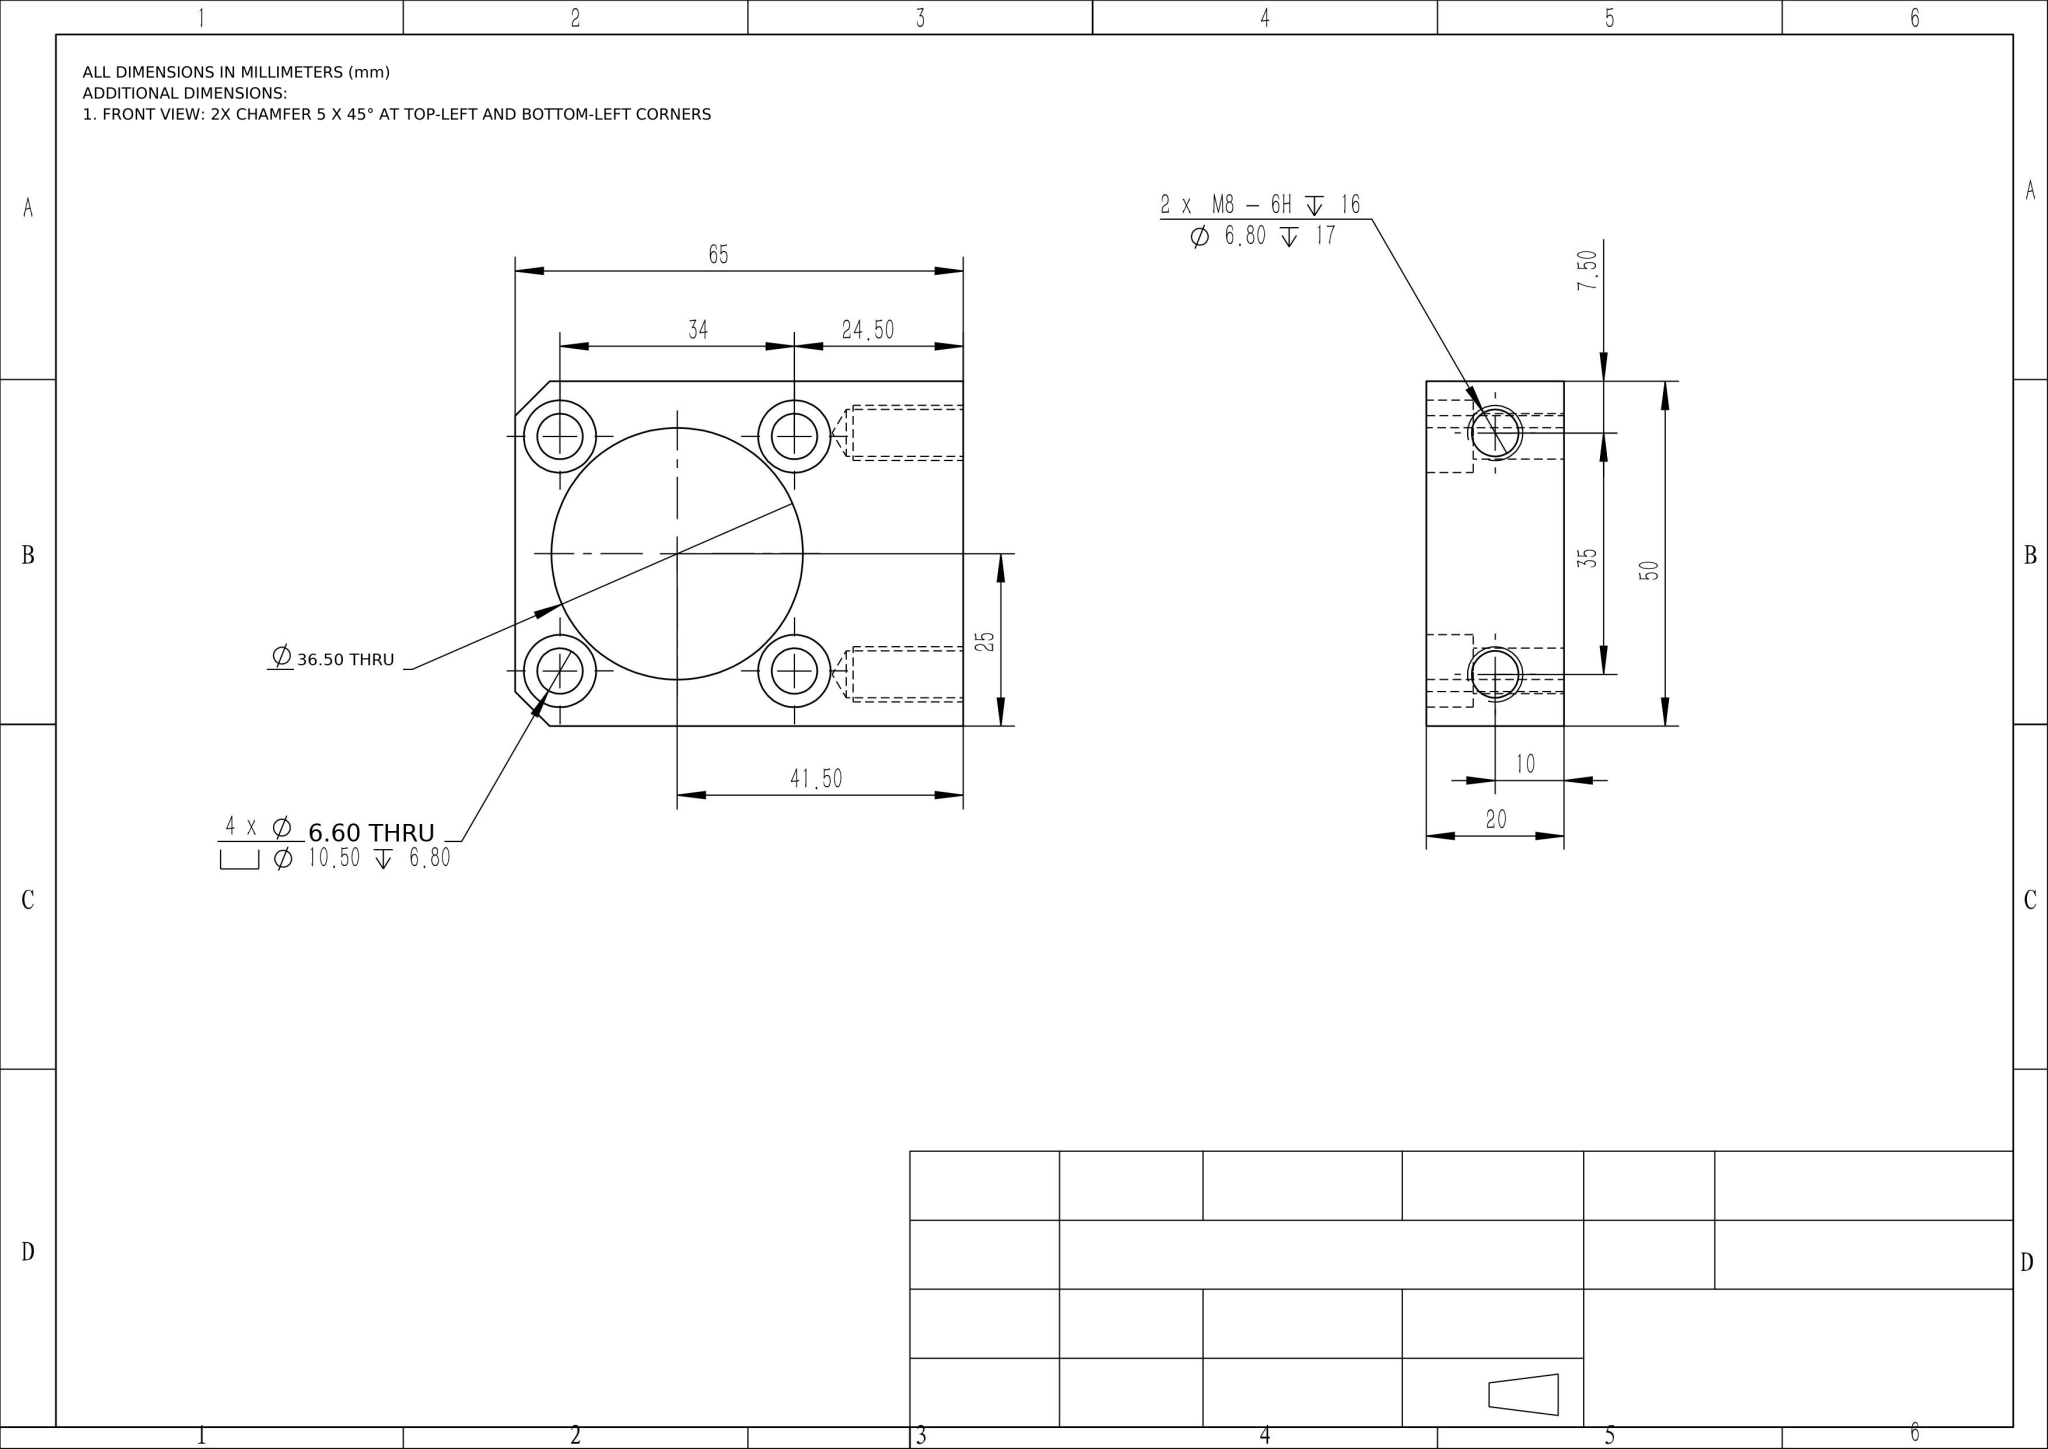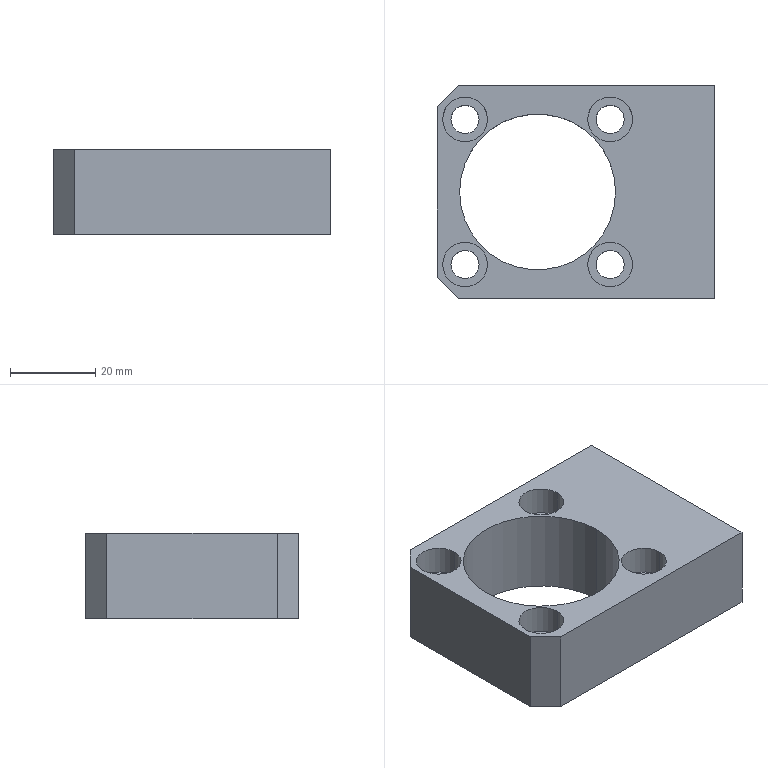Part | NX | mm | 1 solid | 38 faces | box 65 x 50 x 20 mm | volume 38127 mm3 | cylinder 22 | plane 12 | cone 4 | commonest cylinder face diameters 10.5 x8 6.6 x8 6.8 x4 36.5 x2